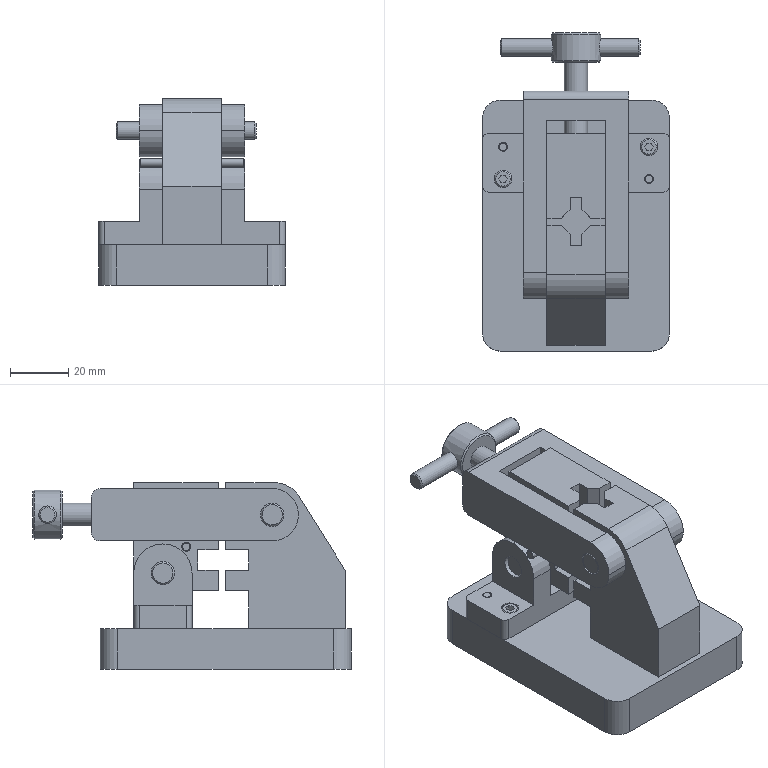Assembly | NX | mm | 13 component files | 13 solids | 181 faces | box 64 x 109 x 64 mm | volume 170915 mm3 | plane 109 | cylinder 51 | cone 21 | commonest cylinder face diameters 3 x12 8 x10 6 x8 20 x6 4 x6 18 x4 12 x4 17 x1
Bill of materials:
unnamed part 1 | 1 |  | Solid straight cylindrical rod with small chamfers at both ends; length roughly 8 times its diameter.
unnamed part 2 | 2 |  | Short solid cylinder with chamfered ends; length roughly 4.5 times its diameter.
unnamed part 3 | 1 |  | Stepped pin made of a plain cylindrical shank and a larger coaxial cylindrical head. The head has a radial through-hole across it and chamfered edges.
unnamed part 4 | 2 |  | Solid cylindrical rod with chamfered ends; length roughly 4.4 times its diameter.
unnamed part 5 | 1 |  | U-shaped fork (clevis-like) block: two parallel flat arms joined by a solid base. The arm ends are rounded and have coaxial through-holes. The base has a through-hole along the fork axis.
unnamed part 6 | 1 |  | Rectangular base plate with rounded corners and an upright block near one edge. The upright has an angled, rounded top profile, a through-hole near the top, a rectangular side notch, and a notch in its top. The plate has four small through-holes near the opposite end.
unnamed part 7 | 1 |  | Rectangular base with rounded corners and two parallel upright lugs. Each lug has a rounded top and a through-hole, and the two holes are coaxial. There are four mounting holes in the base ends, two larger and two smaller.
unnamed part 8 | 1 |  | Prismatic block with one rounded corner. It has a large and a small through-hole near the rounded end, a rectangular notch cut into one side face, and a slot with flared (chamfered) entry on the bottom face.
unnamed part 9 | 1 |  | Long, slender solid cylindrical rod with small chamfers at both ends; length roughly 12 times its diameter.
unnamed part 10 | 2 |  | Fastener-like part: a cylindrical head with a hexagonal socket recess and a chamfered top edge, on a smooth cylindrical shank with a chamfered tip. It resembles a socket head cap screw.
Mates:
1. fix | base 1 component
2. touch align | handle 1 face | threaded_rod 1 face
3. touch align | threaded_rod 1 face | U_bracket 1 face
4. distance | U_bracket 1 face | threaded_rod 1 face
5. distance | handle 1 face | U_bracket 1 face
6. touch align | clamp_block 1 face | base 1 face
7. touch align | clamp_block 1 face | base 1 face
8. touch align | U_bracket 1 face | base 1 face
9. touch align | U_bracket 1 face | base 1 face
10. touch align | bracket 1 face | clamp_block 1 face
11. touch align | bracket 1 face | clamp_block 1 face
12. touch align | base 1 face | bracket 1 face
13. touch align | screw 1 face | bracket 1 face
14. touch align | screw 1 face | bracket 1 face
15. touch align | screw 2 face | bracket 1 face
16. touch align | screw 2 face | bracket 1 face
17. touch align | small_pin 2 face | bracket 1 face
18. touch align | small_pin 2 face | bracket 1 face
19. touch align | small_pin 1 face | bracket 1 face
20. touch align | bracket 1 face | small_pin 1 face
21. touch align | large_pin 1 face | U_bracket 1 face
22. touch align | large_pin 2 face | clamp_block 1 face
23. touch align | large_pin 2 face | bracket 1 face
24. touch align | large_pin 1 face | U_bracket 1 face
25. touch align | support_pin 1 face | clamp_block 1 face
26. distance | support_pin 1 face | clamp_block 1 face